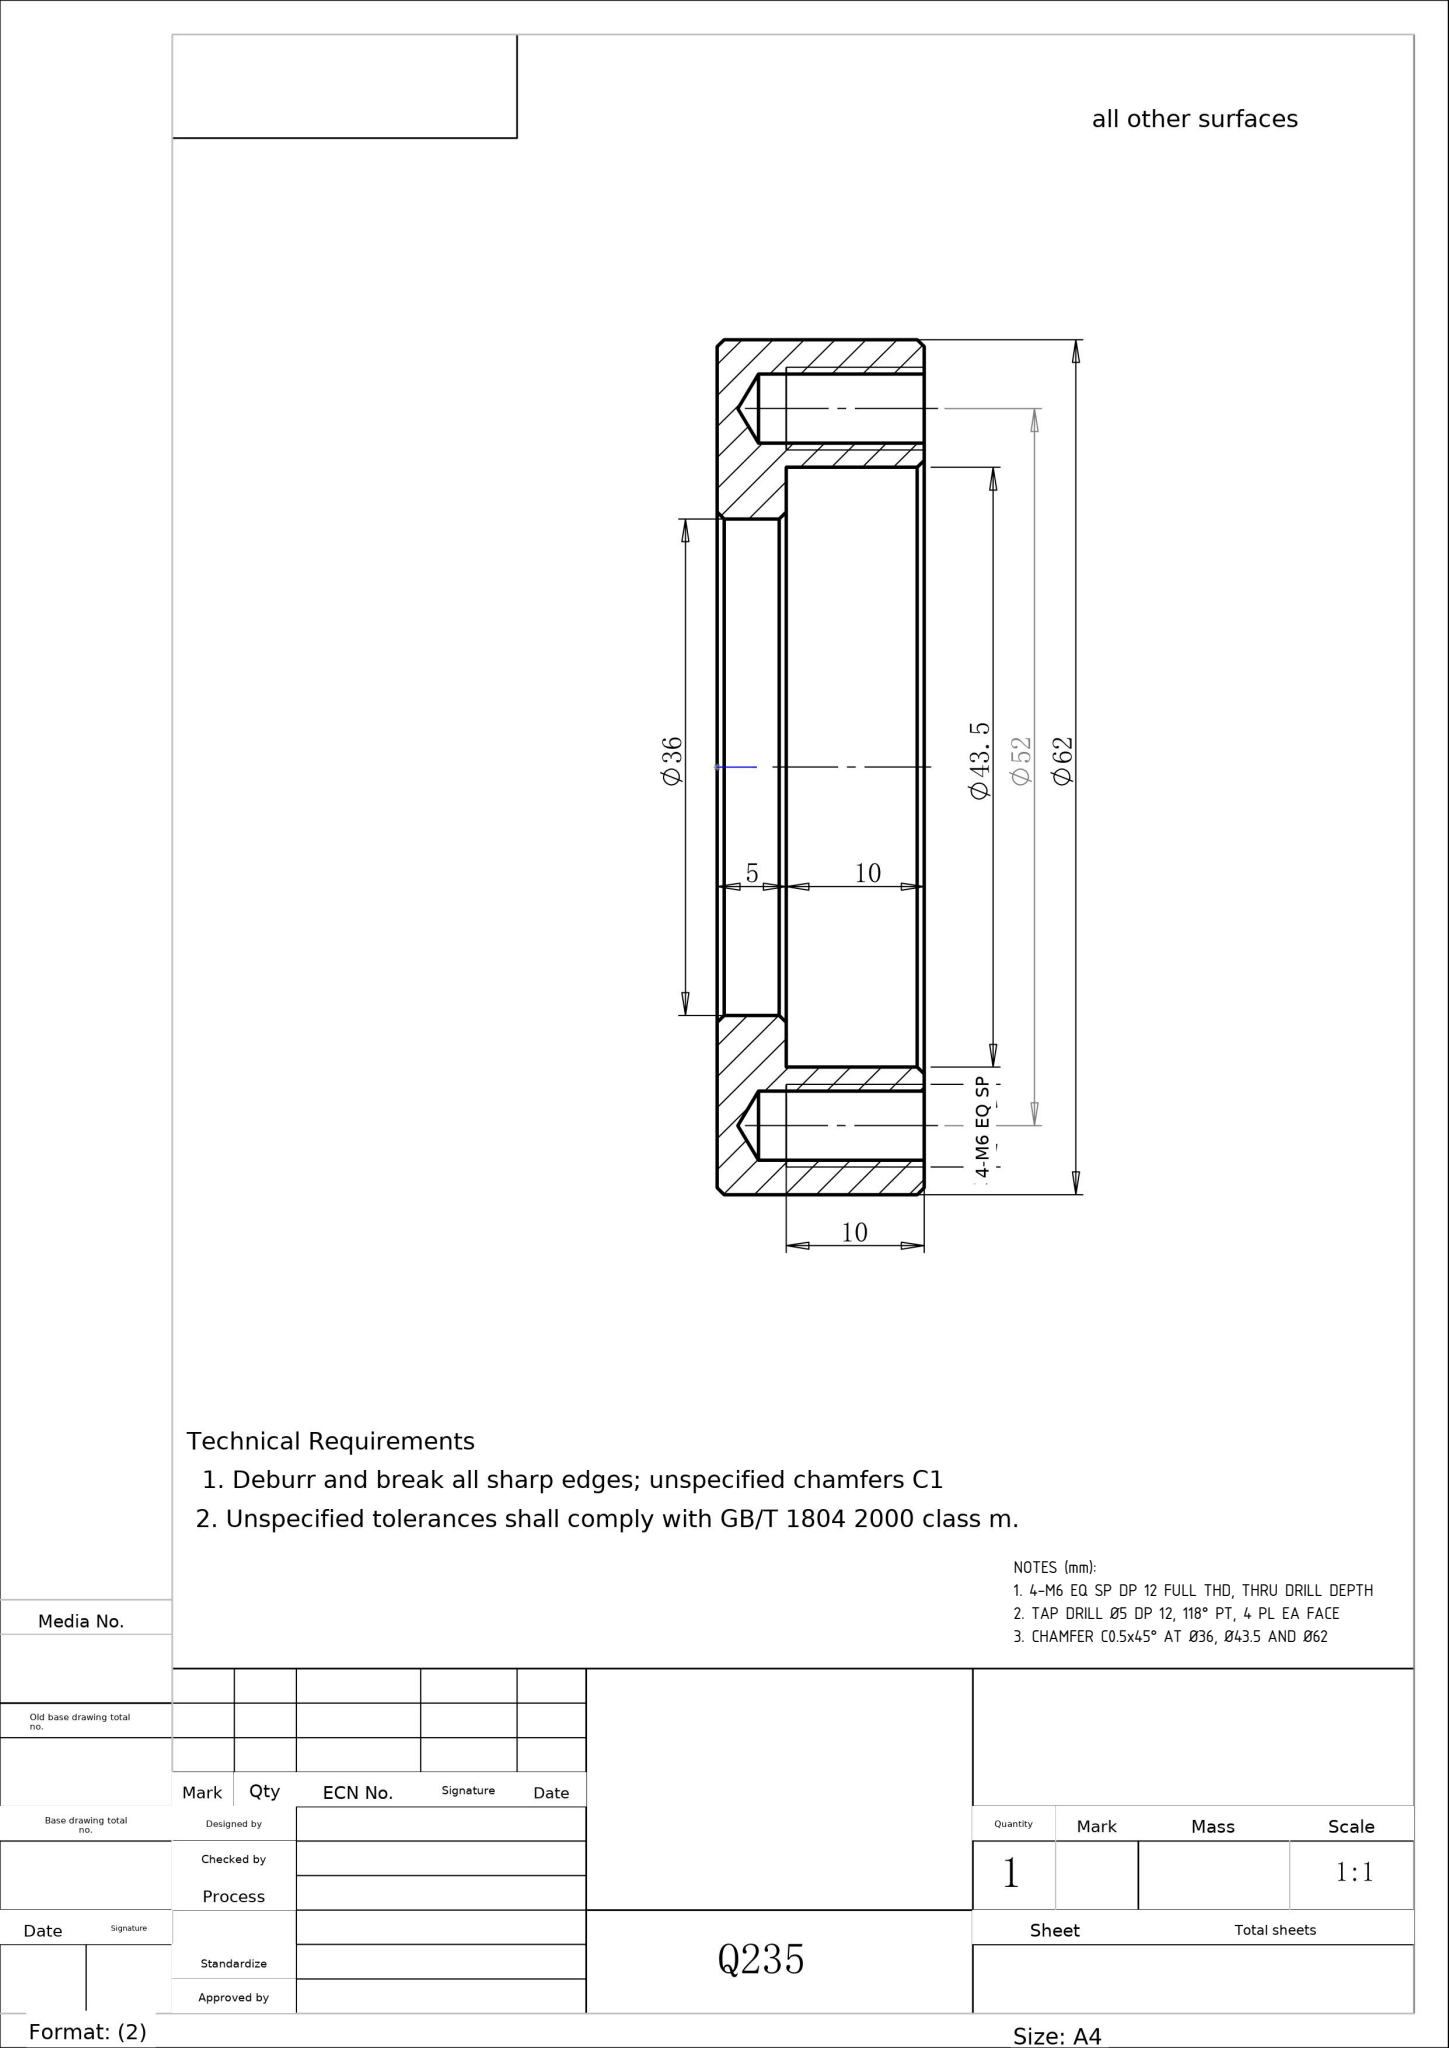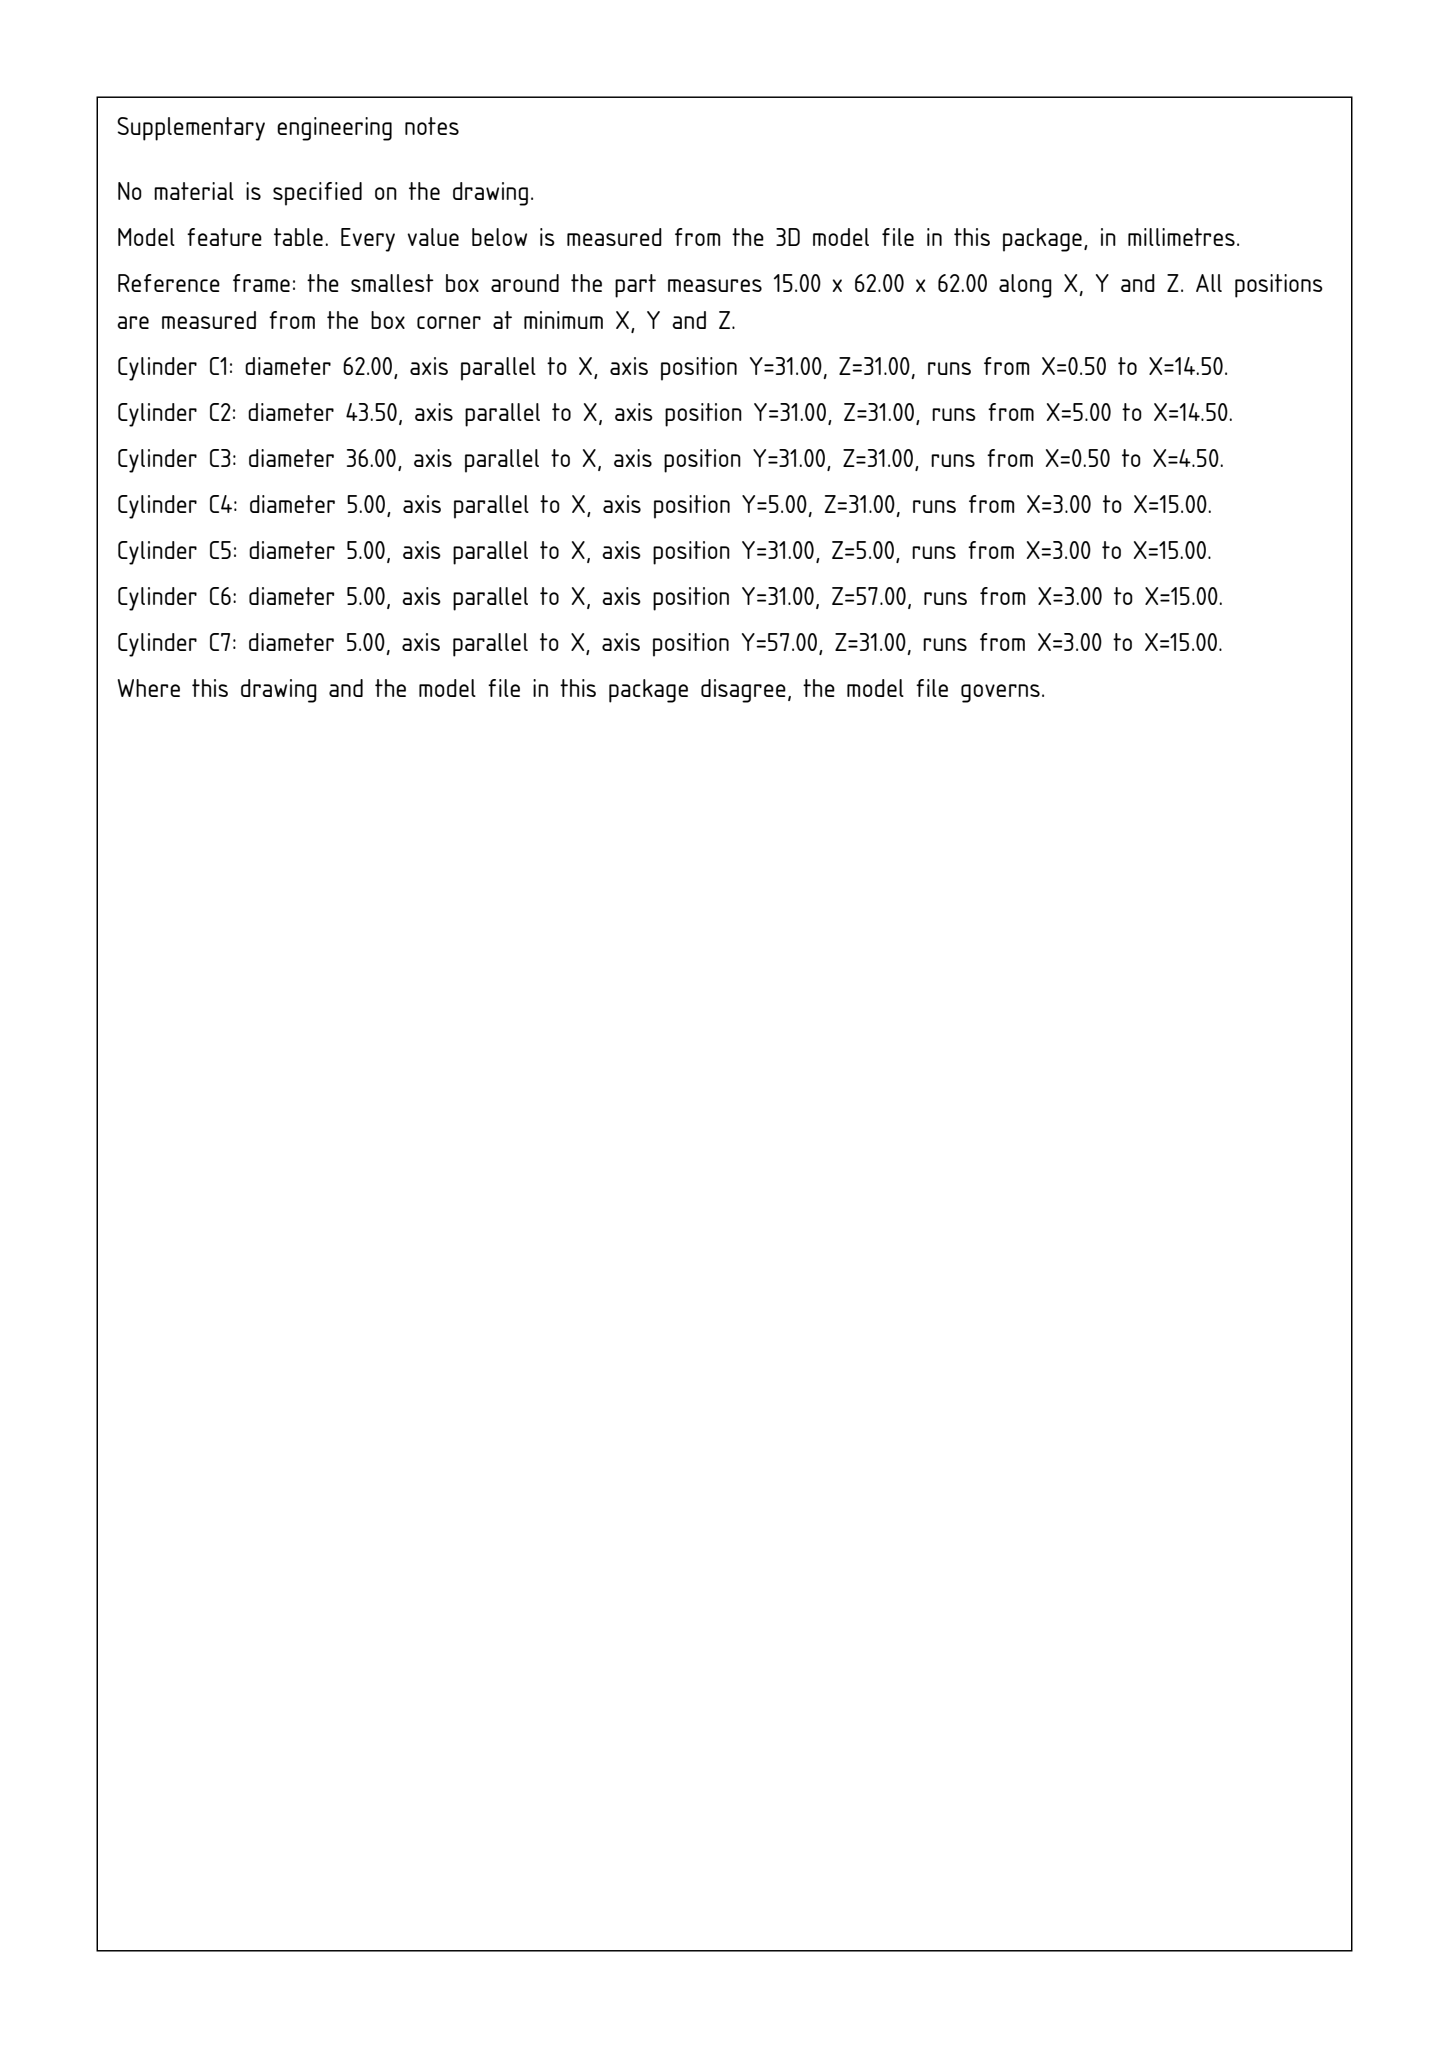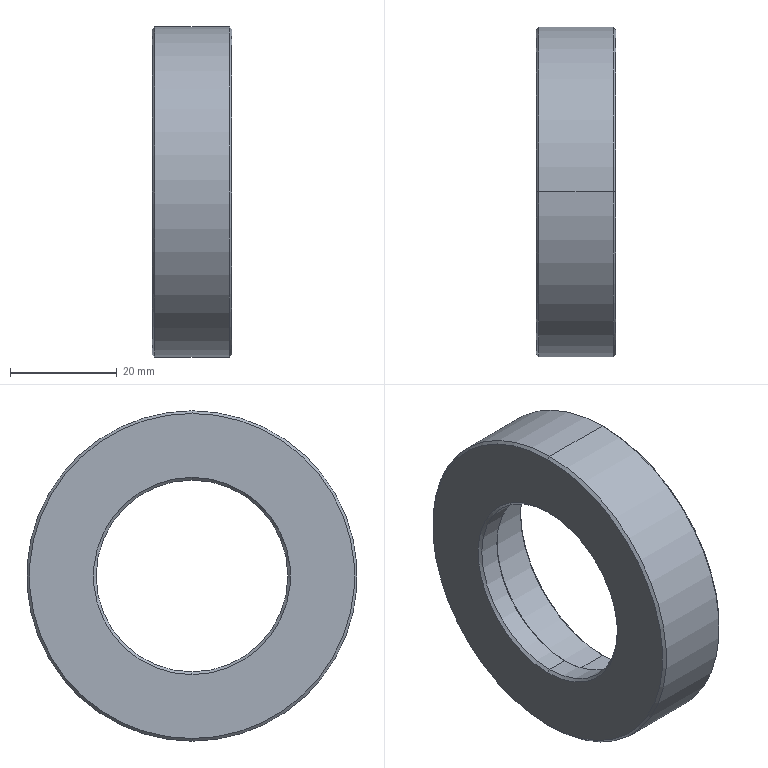Part | SolidWorks | mm | 1 solid | 35 faces | box 15 x 62 x 62 mm | volume 24259 mm3 | cone 18 | cylinder 14 | plane 3 | commonest cylinder face diameters 5 x8 43.5 x2 62 x2 36 x2
Drawing notes:
4-M6 EQ SP DP 12 FULL THD, THRU DRILL DEPTH | from the solid: 4x2 Ø5 cylinders, axis x, length 12.0 from each face, 118° drill point cones
TAP DRILL Ø5 DP 12, 118° PT, 4 PL EA FACE | from the solid: cylinders [5.0,'x',...,12.0] at (5,31),(31,5),(31,57),(57,31); cones 118° ref dia 5.0
CHAMFER C0.5x45° AT Ø36, Ø43.5 AND Ø62 | from the solid: 90° cones ref dia 37.0/36.0 (bore Ø36), 44.5 (bore Ø43.5), 61.0/62.0 (OD Ø62) = 0.5 leg
build123d program:
from build123d import *

# Parameters (mm, degrees)
CHAMFER1_SIZE     = 0.5
CIRPATTERN1_COUNT = 4


with BuildPart() as part:
    # Sketch1 → Revolve1 (revolve)
    with BuildSketch(Plane.XY, mode=Mode.PRIVATE) as revolve1_sk:
        Polygon((5, 21.75), (15, 21.75), (15, 31), (0, 31), (0, 18), (5, 18), align=None)
    revolve(revolve1_sk.sketch.rotate(Axis((0, 0, 0), (1, 0, 0)), 90), axis=Axis((0, 0, 0), (1, 0, 0)))

    # Chamfer1
    chamfer1_edges = [part.edges().sort_by_distance(p)[0] for p in [
        (15, 0, -21.75),
        (15, 0, -31),
        (0, 0, -31),
        (0, 0, -18),
        (5, 0, -18),
    ]]
    chamfer(chamfer1_edges, length=CHAMFER1_SIZE)

    # Sketch2 → M6 Tapped Hole1 (revolve, cut)
    with BuildSketch(Plane(origin=(15, 0, 26), x_dir=(0, 0, -1), z_dir=(0, 1, 0))):
        Polygon((0, 0), (0, 13.502), (2.5, 12), (2.5, 0), align=None)
    m6_tapped_hole1 = revolve(axis=Axis((21.35, 0, 26), (-1, 0, 0)), mode=Mode.SUBTRACT)

    # CirPattern1: M6 Tapped Hole1 ×4 about axis
    cirpattern1_axis = Axis((0, 0, 0), (1, 0, 0))
    for i in range(1, CIRPATTERN1_COUNT):
        add(m6_tapped_hole1.rotate(cirpattern1_axis, i * 360 / CIRPATTERN1_COUNT), mode=Mode.SUBTRACT)


solid = part.part